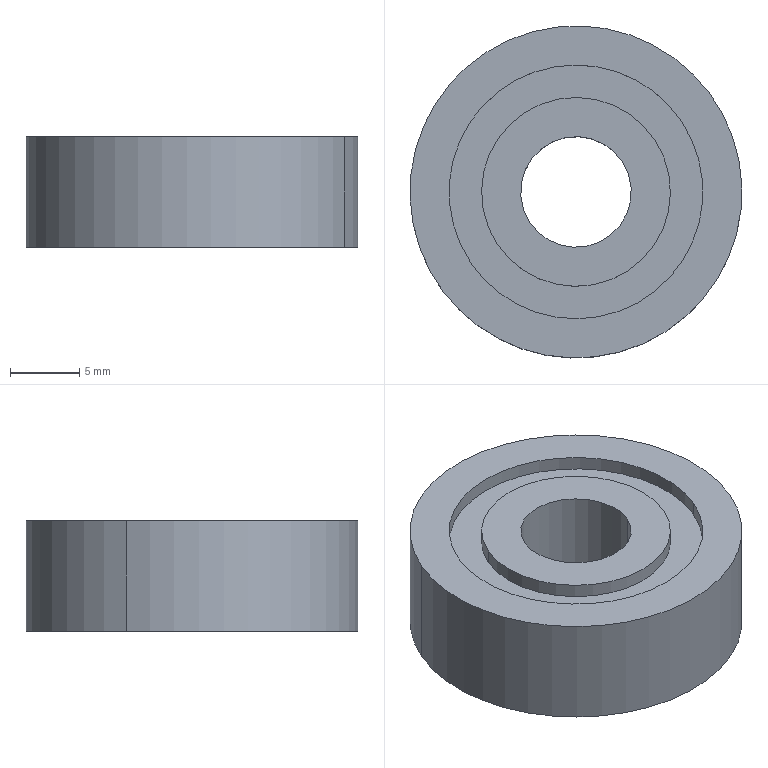Component | SolidWorks | PulleyAssembly-1_Bearing-1 | 1 solid | 18 faces | box 24 x 24 x 8 mm | volume 2981 mm3 | cylinder 12 | plane 6 | commonest cylinder face diameters 13.655 x4 18.345 x4 24 x2 8 x2
build123d program:
from build123d import *


with BuildPart() as part:
    # Sketch1 → Revolve1 (revolve)
    with BuildSketch(Plane(origin=(0, 0, 0), x_dir=(1, 0, 0), z_dir=(0, 1, 0)), mode=Mode.PRIVATE) as revolve1_sk:
        Polygon((4, 4), (6.827, 4), (6.827, 3), (9.173, 3), (9.173, 4), (12, 4), (12, -4), (9.173, -4), (9.173, -3), (6.827, -3), (6.827, -4), (4, -4), align=None)
    revolve(revolve1_sk.sketch.rotate(Axis((0, 0, -4.4), (0, 0, 1)), 180), axis=Axis((0, 0, -4.4), (0, 0, 1)))


solid = part.part

# Placed as in the assembly
solid = solid.moved(Location((-354.55, -345.434, 489.481), (0, 0, 0)))
STEP:
#1=COLOUR_RGB('',0.7922,0.8196,0.9333);
#2=FILL_AREA_STYLE_COLOUR('',#1);
#3=FILL_AREA_STYLE('',(#2));
#4=SURFACE_STYLE_FILL_AREA(#3);
#5=SURFACE_SIDE_STYLE('',(#4));
#6=SURFACE_STYLE_USAGE(.BOTH.,#5);
#7=PRESENTATION_STYLE_ASSIGNMENT((#6));
#8=CARTESIAN_POINT('',(-14.206,-13.493,19.113));
#9=VERTEX_POINT('',#8);
#10=CARTESIAN_POINT('',(-13.712,-13.706,19.113));
#11=VERTEX_POINT('',#10);
#12=CARTESIAN_POINT('',(-13.959,-13.6,19.113));
#13=DIRECTION('',(-0.,0.,1.));
#14=DIRECTION('',(-0.9185,0.3954,0.));
#15=AXIS2_PLACEMENT_3D('',#12,#13,#14);
#16=CIRCLE('',#15,0.2688);
#17=EDGE_CURVE('',#9,#11,#16,.T.);
#18=ORIENTED_EDGE('',*,*,#17,.T.);
#19=CARTESIAN_POINT('',(-13.712,-13.706,19.153));
#20=VERTEX_POINT('',#19);
#21=CARTESIAN_POINT('',(-13.712,-13.706,19.444));
#22=DIRECTION('',(-0.,0.,1.));
#23=VECTOR('',#22,39.37);
#24=LINE('',#21,#23);
#25=EDGE_CURVE('',#11,#20,#24,.T.);
#26=ORIENTED_EDGE('',*,*,#25,.T.);
#27=CARTESIAN_POINT('',(-14.206,-13.493,19.153));
#28=VERTEX_POINT('',#27);
#29=CARTESIAN_POINT('',(-13.959,-13.6,19.153));
#30=DIRECTION('',(-0.,0.,1.));
#31=DIRECTION('',(-0.9185,0.3954,0.));
#32=AXIS2_PLACEMENT_3D('',#29,#30,#31);
#33=CIRCLE('',#32,0.2688);
#34=EDGE_CURVE('',#28,#20,#33,.T.);
#35=ORIENTED_EDGE('',*,*,#34,.F.);
#36=CARTESIAN_POINT('',(-14.206,-13.493,19.444));
#37=DIRECTION('',(-0.,0.,1.));
#38=VECTOR('',#37,39.37);
#39=LINE('',#36,#38);
#40=EDGE_CURVE('',#9,#28,#39,.T.);
#41=ORIENTED_EDGE('',*,*,#40,.F.);
#42=EDGE_LOOP('',(#18,#26,#35,#41));
#43=FACE_OUTER_BOUND('',#42,.T.);
#44=CARTESIAN_POINT('',(-13.959,-13.6,19.444));
#45=DIRECTION('',(-0.,0.,1.));
#46=DIRECTION('',(-0.9185,0.3954,0.));
#47=AXIS2_PLACEMENT_3D('',#44,#45,#46);
#48=CYLINDRICAL_SURFACE('',#47,0.2688);
#49=ADVANCED_FACE('',(#43),#48,.T.);
#50=CARTESIAN_POINT('',(-13.627,-13.743,19.113));
#51=VERTEX_POINT('',#50);
#52=CARTESIAN_POINT('',(-14.29,-13.457,19.113));
#53=VERTEX_POINT('',#52);
#54=CARTESIAN_POINT('',(-13.959,-13.6,19.113));
#55=DIRECTION('',(-0.,0.,1.));
#56=DIRECTION('',(-0.9185,0.3954,0.));
#57=AXIS2_PLACEMENT_3D('',#54,#55,#56);
#58=CIRCLE('',#57,0.3611);
#59=EDGE_CURVE('',#51,#53,#58,.T.);
#60=ORIENTED_EDGE('',*,*,#59,.F.);
#61=CARTESIAN_POINT('',(-13.627,-13.743,19.153));
#62=VERTEX_POINT('',#61);
#63=CARTESIAN_POINT('',(-13.627,-13.743,19.444));
#64=DIRECTION('',(-0.,0.,1.));
#65=VECTOR('',#64,39.37);
#66=LINE('',#63,#65);
#67=EDGE_CURVE('',#51,#62,#66,.T.);
#68=ORIENTED_EDGE('',*,*,#67,.T.);
#69=CARTESIAN_POINT('',(-14.29,-13.457,19.153));
#70=VERTEX_POINT('',#69);
#71=CARTESIAN_POINT('',(-13.959,-13.6,19.153));
#72=DIRECTION('',(-0.,0.,1.));
#73=DIRECTION('',(-0.9185,0.3954,0.));
#74=AXIS2_PLACEMENT_3D('',#71,#72,#73);
#75=CIRCLE('',#74,0.3611);
#76=EDGE_CURVE('',#62,#70,#75,.T.);
#77=ORIENTED_EDGE('',*,*,#76,.T.);
#78=CARTESIAN_POINT('',(-14.29,-13.457,19.444));
#79=DIRECTION('',(-0.,0.,1.));
#80=VECTOR('',#79,39.37);
#81=LINE('',#78,#80);
#82=EDGE_CURVE('',#53,#70,#81,.T.);
#83=ORIENTED_EDGE('',*,*,#82,.F.);
#84=EDGE_LOOP('',(#60,#68,#77,#83));
#85=FACE_OUTER_BOUND('',#84,.T.);
#86=CARTESIAN_POINT('',(-13.959,-13.6,19.444));
#87=DIRECTION('',(-0.,0.,1.));
#88=DIRECTION('',(-0.9185,0.3954,0.));
#89=AXIS2_PLACEMENT_3D('',#86,#87,#88);
#90=CYLINDRICAL_SURFACE('',#89,0.3611);
#91=ADVANCED_FACE('',(#85),#90,.F.);
#92=CARTESIAN_POINT('',(-14.393,-13.413,19.113));
#93=VERTEX_POINT('',#92);
#94=CARTESIAN_POINT('',(-13.525,-13.787,19.113));
#95=VERTEX_POINT('',#94);
#96=CARTESIAN_POINT('',(-13.959,-13.6,19.113));
#97=DIRECTION('',(-0.,0.,1.));
#98=DIRECTION('',(-0.9185,0.3954,0.));
#99=AXIS2_PLACEMENT_3D('',#96,#97,#98);
#100=CIRCLE('',#99,0.4724);
#101=EDGE_CURVE('',#93,#95,#100,.T.);
#102=ORIENTED_EDGE('',*,*,#101,.T.);
#103=CARTESIAN_POINT('',(-13.525,-13.787,19.428));
#104=VERTEX_POINT('',#103);
#105=CARTESIAN_POINT('',(-13.525,-13.787,19.444));
#106=DIRECTION('',(-0.,0.,1.));
#107=VECTOR('',#106,39.37);
#108=LINE('',#105,#107);
#109=EDGE_CURVE('',#95,#104,#108,.T.);
#110=ORIENTED_EDGE('',*,*,#109,.T.);
#111=CARTESIAN_POINT('',(-14.393,-13.413,19.428));
#112=VERTEX_POINT('',#111);
#113=CARTESIAN_POINT('',(-13.959,-13.6,19.428));
#114=DIRECTION('',(-0.,0.,1.));
#115=DIRECTION('',(-0.9185,0.3954,0.));
#116=AXIS2_PLACEMENT_3D('',#113,#114,#115);
#117=CIRCLE('',#116,0.4724);
#118=EDGE_CURVE('',#112,#104,#117,.T.);
#119=ORIENTED_EDGE('',*,*,#118,.F.);
#120=CARTESIAN_POINT('',(-14.393,-13.413,19.444));
#121=DIRECTION('',(-0.,0.,1.));
#122=VECTOR('',#121,39.37);
#123=LINE('',#120,#122);
#124=EDGE_CURVE('',#93,#112,#123,.T.);
#125=ORIENTED_EDGE('',*,*,#124,.F.);
#126=EDGE_LOOP('',(#102,#110,#119,#125));
#127=FACE_OUTER_BOUND('',#126,.T.);
#128=CARTESIAN_POINT('',(-13.959,-13.6,19.444));
#129=DIRECTION('',(-0.,0.,1.));
#130=DIRECTION('',(-0.9185,0.3954,0.));
#131=AXIS2_PLACEMENT_3D('',#128,#129,#130);
#132=CYLINDRICAL_SURFACE('',#131,0.4724);
#133=ADVANCED_FACE('',(#127),#132,.T.);
#134=CARTESIAN_POINT('',(-13.627,-13.743,19.389));
#135=VERTEX_POINT('',#134);
#136=CARTESIAN_POINT('',(-14.29,-13.457,19.389));
#137=VERTEX_POINT('',#136);
#138=CARTESIAN_POINT('',(-13.959,-13.6,19.389));
#139=DIRECTION('',(-0.,0.,1.));
#140=DIRECTION('',(-0.9185,0.3954,0.));
#141=AXIS2_PLACEMENT_3D('',#138,#139,#140);
#142=CIRCLE('',#141,0.3611);
#143=EDGE_CURVE('',#135,#137,#142,.T.);
#144=ORIENTED_EDGE('',*,*,#143,.F.);
#145=CARTESIAN_POINT('',(-13.627,-13.743,19.428));
#146=VERTEX_POINT('',#145);
#147=CARTESIAN_POINT('',(-13.627,-13.743,19.444));
#148=DIRECTION('',(-0.,0.,1.));
#149=VECTOR('',#148,39.37);
#150=LINE('',#147,#149);
#151=EDGE_CURVE('',#135,#146,#150,.T.);
#152=ORIENTED_EDGE('',*,*,#151,.T.);
#153=CARTESIAN_POINT('',(-14.29,-13.457,19.428));
#154=VERTEX_POINT('',#153);
#155=CARTESIAN_POINT('',(-13.959,-13.6,19.428));
#156=DIRECTION('',(-0.,0.,1.));
#157=DIRECTION('',(-0.9185,0.3954,0.));
#158=AXIS2_PLACEMENT_3D('',#155,#156,#157);
#159=CIRCLE('',#158,0.3611);
#160=EDGE_CURVE('',#146,#154,#159,.T.);
#161=ORIENTED_EDGE('',*,*,#160,.T.);
#162=CARTESIAN_POINT('',(-14.29,-13.457,19.444));
#163=DIRECTION('',(-0.,0.,1.));
#164=VECTOR('',#163,39.37);
#165=LINE('',#162,#164);
#166=EDGE_CURVE('',#137,#154,#165,.T.);
#167=ORIENTED_EDGE('',*,*,#166,.F.);
#168=EDGE_LOOP('',(#144,#152,#161,#167));
#169=FACE_OUTER_BOUND('',#168,.T.);
#170=CARTESIAN_POINT('',(-13.959,-13.6,19.444));
#171=DIRECTION('',(-0.,0.,1.));
#172=DIRECTION('',(-0.9185,0.3954,0.));
#173=AXIS2_PLACEMENT_3D('',#170,#171,#172);
#174=CYLINDRICAL_SURFACE('',#173,0.3611);
#175=ADVANCED_FACE('',(#169),#174,.F.);
#176=CARTESIAN_POINT('',(-14.206,-13.493,19.389));
#177=VERTEX_POINT('',#176);
#178=CARTESIAN_POINT('',(-13.712,-13.706,19.389));
#179=VERTEX_POINT('',#178);
#180=CARTESIAN_POINT('',(-13.959,-13.6,19.389));
#181=DIRECTION('',(-0.,0.,1.));
#182=DIRECTION('',(-0.9185,0.3954,0.));
#183=AXIS2_PLACEMENT_3D('',#180,#181,#182);
#184=CIRCLE('',#183,0.2688);
#185=EDGE_CURVE('',#177,#179,#184,.T.);
#186=ORIENTED_EDGE('',*,*,#185,.T.);
#187=CARTESIAN_POINT('',(-13.712,-13.706,19.428));
#188=VERTEX_POINT('',#187);
#189=CARTESIAN_POINT('',(-13.712,-13.706,19.444));
#190=DIRECTION('',(-0.,0.,1.));
#191=VECTOR('',#190,39.37);
#192=LINE('',#189,#191);
#193=EDGE_CURVE('',#179,#188,#192,.T.);
#194=ORIENTED_EDGE('',*,*,#193,.T.);
#195=CARTESIAN_POINT('',(-14.206,-13.493,19.428));
#196=VERTEX_POINT('',#195);
#197=CARTESIAN_POINT('',(-13.959,-13.6,19.428));
#198=DIRECTION('',(-0.,0.,1.));
#199=DIRECTION('',(-0.9185,0.3954,0.));
#200=AXIS2_PLACEMENT_3D('',#197,#198,#199);
#201=CIRCLE('',#200,0.2688);
#202=EDGE_CURVE('',#196,#188,#201,.T.);
#203=ORIENTED_EDGE('',*,*,#202,.F.);
#204=CARTESIAN_POINT('',(-14.206,-13.493,19.444));
#205=DIRECTION('',(-0.,0.,1.));
#206=VECTOR('',#205,39.37);
#207=LINE('',#204,#206);
#208=EDGE_CURVE('',#177,#196,#207,.T.);
#209=ORIENTED_EDGE('',*,*,#208,.F.);
#210=EDGE_LOOP('',(#186,#194,#203,#209));
#211=FACE_OUTER_BOUND('',#210,.T.);
#212=CARTESIAN_POINT('',(-13.959,-13.6,19.444));
#213=DIRECTION('',(-0.,0.,1.));
#214=DIRECTION('',(-0.9185,0.3954,0.));
#215=AXIS2_PLACEMENT_3D('',#212,#213,#214);
#216=CYLINDRICAL_SURFACE('',#215,0.2688);
#217=ADVANCED_FACE('',(#211),#216,.T.);
#218=CARTESIAN_POINT('',(-13.814,-13.662,19.113));
#219=VERTEX_POINT('',#218);
#220=CARTESIAN_POINT('',(-14.103,-13.537,19.113));
#221=VERTEX_POINT('',#220);
#222=CARTESIAN_POINT('',(-13.959,-13.6,19.113));
#223=DIRECTION('',(-0.,0.,1.));
#224=DIRECTION('',(-0.9185,0.3954,0.));
#225=AXIS2_PLACEMENT_3D('',#222,#223,#224);
#226=CIRCLE('',#225,0.1575);
#227=EDGE_CURVE('',#219,#221,#226,.T.);
#228=ORIENTED_EDGE('',*,*,#227,.F.);
#229=CARTESIAN_POINT('',(-13.814,-13.662,19.428));
#230=VERTEX_POINT('',#229);
#231=CARTESIAN_POINT('',(-13.814,-13.662,19.444));
#232=DIRECTION('',(-0.,0.,1.));
#233=VECTOR('',#232,39.37);
#234=LINE('',#231,#233);
#235=EDGE_CURVE('',#219,#230,#234,.T.);
#236=ORIENTED_EDGE('',*,*,#235,.T.);
#237=CARTESIAN_POINT('',(-14.103,-13.537,19.428));
#238=VERTEX_POINT('',#237);
#239=CARTESIAN_POINT('',(-13.959,-13.6,19.428));
#240=DIRECTION('',(-0.,0.,1.));
#241=DIRECTION('',(-0.9185,0.3954,0.));
#242=AXIS2_PLACEMENT_3D('',#239,#240,#241);
#243=CIRCLE('',#242,0.1575);
#244=EDGE_CURVE('',#230,#238,#243,.T.);
#245=ORIENTED_EDGE('',*,*,#244,.T.);
#246=CARTESIAN_POINT('',(-14.103,-13.537,19.444));
#247=DIRECTION('',(-0.,0.,1.));
#248=VECTOR('',#247,39.37);
#249=LINE('',#246,#248);
#250=EDGE_CURVE('',#221,#238,#249,.T.);
#251=ORIENTED_EDGE('',*,*,#250,.F.);
#252=EDGE_LOOP('',(#228,#236,#245,#251));
#253=FACE_OUTER_BOUND('',#252,.T.);
#254=CARTESIAN_POINT('',(-13.959,-13.6,19.444));
#255=DIRECTION('',(-0.,0.,1.));
#256=DIRECTION('',(-0.9185,0.3954,0.));
#257=AXIS2_PLACEMENT_3D('',#254,#255,#256);
#258=CYLINDRICAL_SURFACE('',#257,0.1575);
#259=ADVANCED_FACE('',(#253),#258,.F.);
#260=ORIENTED_EDGE('',*,*,#235,.F.);
#261=CARTESIAN_POINT('',(-13.959,-13.6,19.113));
#262=DIRECTION('',(-0.,0.,1.));
#263=DIRECTION('',(-0.9185,0.3954,0.));
#264=AXIS2_PLACEMENT_3D('',#261,#262,#263);
#265=CIRCLE('',#264,0.1575);
#266=EDGE_CURVE('',#221,#219,#265,.T.);
#267=ORIENTED_EDGE('',*,*,#266,.F.);
#268=ORIENTED_EDGE('',*,*,#250,.T.);
#269=CARTESIAN_POINT('',(-13.959,-13.6,19.428));
#270=DIRECTION('',(-0.,0.,1.));
#271=DIRECTION('',(-0.9185,0.3954,0.));
#272=AXIS2_PLACEMENT_3D('',#269,#270,#271);
#273=CIRCLE('',#272,0.1575);
#274=EDGE_CURVE('',#238,#230,#273,.T.);
#275=ORIENTED_EDGE('',*,*,#274,.T.);
#276=EDGE_LOOP('',(#260,#267,#268,#275));
#277=FACE_OUTER_BOUND('',#276,.T.);
#278=CARTESIAN_POINT('',(-13.959,-13.6,19.444));
#279=DIRECTION('',(-0.,0.,1.));
#280=DIRECTION('',(-0.9185,0.3954,0.));
#281=AXIS2_PLACEMENT_3D('',#278,#279,#280);
#282=CYLINDRICAL_SURFACE('',#281,0.1575);
#283=ADVANCED_FACE('',(#277),#282,.F.);
#284=ORIENTED_EDGE('',*,*,#274,.F.);
#285=ORIENTED_EDGE('',*,*,#244,.F.);
#286=EDGE_LOOP('',(#284,#285));
#287=FACE_BOUND('',#286,.T.);
#288=ORIENTED_EDGE('',*,*,#202,.T.);
#289=CARTESIAN_POINT('',(-13.959,-13.6,19.428));
#290=DIRECTION('',(-0.,0.,1.));
#291=DIRECTION('',(-0.9185,0.3954,0.));
#292=AXIS2_PLACEMENT_3D('',#289,#290,#291);
#293=CIRCLE('',#292,0.2688);
#294=EDGE_CURVE('',#188,#196,#293,.T.);
#295=ORIENTED_EDGE('',*,*,#294,.T.);
#296=EDGE_LOOP('',(#288,#295));
#297=FACE_OUTER_BOUND('',#296,.T.);
#298=CARTESIAN_POINT('',(-13.814,-13.662,19.428));
#299=DIRECTION('',(0.,-0.,-1.));
#300=DIRECTION('',(0.9185,-0.3954,0.));
#301=AXIS2_PLACEMENT_3D('',#298,#299,#300);
#302=PLANE('',#301);
#303=ADVANCED_FACE('',(#287,#297),#302,.F.);
#304=ORIENTED_EDGE('',*,*,#193,.F.);
#305=CARTESIAN_POINT('',(-13.959,-13.6,19.389));
#306=DIRECTION('',(-0.,0.,1.));
#307=DIRECTION('',(-0.9185,0.3954,0.));
#308=AXIS2_PLACEMENT_3D('',#305,#306,#307);
#309=CIRCLE('',#308,0.2688);
#310=EDGE_CURVE('',#179,#177,#309,.T.);
#311=ORIENTED_EDGE('',*,*,#310,.T.);
#312=ORIENTED_EDGE('',*,*,#208,.T.);
#313=ORIENTED_EDGE('',*,*,#294,.F.);
#314=EDGE_LOOP('',(#304,#311,#312,#313));
#315=FACE_OUTER_BOUND('',#314,.T.);
#316=CARTESIAN_POINT('',(-13.959,-13.6,19.444));
#317=DIRECTION('',(-0.,0.,1.));
#318=DIRECTION('',(-0.9185,0.3954,0.));
#319=AXIS2_PLACEMENT_3D('',#316,#317,#318);
#320=CYLINDRICAL_SURFACE('',#319,0.2688);
#321=ADVANCED_FACE('',(#315),#320,.T.);
#322=ORIENTED_EDGE('',*,*,#185,.F.);
#323=ORIENTED_EDGE('',*,*,#310,.F.);
#324=EDGE_LOOP('',(#322,#323));
#325=FACE_BOUND('',#324,.T.);
#326=CARTESIAN_POINT('',(-13.959,-13.6,19.389));
#327=DIRECTION('',(-0.,0.,1.));
#328=DIRECTION('',(-0.9185,0.3954,0.));
#329=AXIS2_PLACEMENT_3D('',#326,#327,#328);
#330=CIRCLE('',#329,0.3611);
#331=EDGE_CURVE('',#137,#135,#330,.T.);
#332=ORIENTED_EDGE('',*,*,#331,.T.);
#333=ORIENTED_EDGE('',*,*,#143,.T.);
#334=EDGE_LOOP('',(#332,#333));
#335=FACE_OUTER_BOUND('',#334,.T.);
#336=CARTESIAN_POINT('',(-13.627,-13.743,19.389));
#337=DIRECTION('',(0.,-0.,-1.));
#338=DIRECTION('',(0.9185,-0.3954,0.));
#339=AXIS2_PLACEMENT_3D('',#336,#337,#338);
#340=PLANE('',#339);
#341=ADVANCED_FACE('',(#325,#335),#340,.F.);
#342=ORIENTED_EDGE('',*,*,#151,.F.);
#343=ORIENTED_EDGE('',*,*,#331,.F.);
#344=ORIENTED_EDGE('',*,*,#166,.T.);
#345=CARTESIAN_POINT('',(-13.959,-13.6,19.428));
#346=DIRECTION('',(-0.,0.,1.));
#347=DIRECTION('',(-0.9185,0.3954,0.));
#348=AXIS2_PLACEMENT_3D('',#345,#346,#347);
#349=CIRCLE('',#348,0.3611);
#350=EDGE_CURVE('',#154,#146,#349,.T.);
#351=ORIENTED_EDGE('',*,*,#350,.T.);
#352=EDGE_LOOP('',(#342,#343,#344,#351));
#353=FACE_OUTER_BOUND('',#352,.T.);
#354=CARTESIAN_POINT('',(-13.959,-13.6,19.444));
#355=DIRECTION('',(-0.,0.,1.));
#356=DIRECTION('',(-0.9185,0.3954,0.));
#357=AXIS2_PLACEMENT_3D('',#354,#355,#356);
#358=CYLINDRICAL_SURFACE('',#357,0.3611);
#359=ADVANCED_FACE('',(#353),#358,.F.);
#360=ORIENTED_EDGE('',*,*,#350,.F.);
#361=ORIENTED_EDGE('',*,*,#160,.F.);
#362=EDGE_LOOP('',(#360,#361));
#363=FACE_BOUND('',#362,.T.);
#364=ORIENTED_EDGE('',*,*,#118,.T.);
#365=CARTESIAN_POINT('',(-13.959,-13.6,19.428));
#366=DIRECTION('',(-0.,0.,1.));
#367=DIRECTION('',(-0.9185,0.3954,0.));
#368=AXIS2_PLACEMENT_3D('',#365,#366,#367);
#369=CIRCLE('',#368,0.4724);
#370=EDGE_CURVE('',#104,#112,#369,.T.);
#371=ORIENTED_EDGE('',*,*,#370,.T.);
#372=EDGE_LOOP('',(#364,#371));
#373=FACE_OUTER_BOUND('',#372,.T.);
#374=CARTESIAN_POINT('',(-13.627,-13.743,19.428));
#375=DIRECTION('',(0.,-0.,-1.));
#376=DIRECTION('',(0.9185,-0.3954,0.));
#377=AXIS2_PLACEMENT_3D('',#374,#375,#376);
#378=PLANE('',#377);
#379=ADVANCED_FACE('',(#363,#373),#378,.F.);
#380=ORIENTED_EDGE('',*,*,#109,.F.);
#381=CARTESIAN_POINT('',(-13.959,-13.6,19.113));
#382=DIRECTION('',(-0.,0.,1.));
#383=DIRECTION('',(-0.9185,0.3954,0.));
#384=AXIS2_PLACEMENT_3D('',#381,#382,#383);
#385=CIRCLE('',#384,0.4724);
#386=EDGE_CURVE('',#95,#93,#385,.T.);
#387=ORIENTED_EDGE('',*,*,#386,.T.);
#388=ORIENTED_EDGE('',*,*,#124,.T.);
#389=ORIENTED_EDGE('',*,*,#370,.F.);
#390=EDGE_LOOP('',(#380,#387,#388,#389));
#391=FACE_OUTER_BOUND('',#390,.T.);
#392=CARTESIAN_POINT('',(-13.959,-13.6,19.444));
#393=DIRECTION('',(-0.,0.,1.));
#394=DIRECTION('',(-0.9185,0.3954,0.));
#395=AXIS2_PLACEMENT_3D('',#392,#393,#394);
#396=CYLINDRICAL_SURFACE('',#395,0.4724);
#397=ADVANCED_FACE('',(#391),#396,.T.);
#398=ORIENTED_EDGE('',*,*,#101,.F.);
#399=ORIENTED_EDGE('',*,*,#386,.F.);
#400=EDGE_LOOP('',(#398,#399));
#401=FACE_OUTER_BOUND('',#400,.T.);
#402=CARTESIAN_POINT('',(-13.959,-13.6,19.113));
#403=DIRECTION('',(-0.,0.,1.));
#404=DIRECTION('',(-0.9185,0.3954,0.));
#405=AXIS2_PLACEMENT_3D('',#402,#403,#404);
#406=CIRCLE('',#405,0.3611);
#407=EDGE_CURVE('',#53,#51,#406,.T.);
#408=ORIENTED_EDGE('',*,*,#407,.T.);
#409=ORIENTED_EDGE('',*,*,#59,.T.);
#410=EDGE_LOOP('',(#408,#409));
#411=FACE_BOUND('',#410,.T.);
#412=CARTESIAN_POINT('',(-13.525,-13.787,19.113));
#413=DIRECTION('',(-0.,0.,1.));
#414=DIRECTION('',(-0.9185,0.3954,-0.));
#415=AXIS2_PLACEMENT_3D('',#412,#413,#414);
#416=PLANE('',#415);
#417=ADVANCED_FACE('',(#401,#411),#416,.F.);
#418=ORIENTED_EDGE('',*,*,#67,.F.);
#419=ORIENTED_EDGE('',*,*,#407,.F.);
#420=ORIENTED_EDGE('',*,*,#82,.T.);
#421=CARTESIAN_POINT('',(-13.959,-13.6,19.153));
#422=DIRECTION('',(-0.,0.,1.));
#423=DIRECTION('',(-0.9185,0.3954,0.));
#424=AXIS2_PLACEMENT_3D('',#421,#422,#423);
#425=CIRCLE('',#424,0.3611);
#426=EDGE_CURVE('',#70,#62,#425,.T.);
#427=ORIENTED_EDGE('',*,*,#426,.T.);
#428=EDGE_LOOP('',(#418,#419,#420,#427));
#429=FACE_OUTER_BOUND('',#428,.T.);
#430=CARTESIAN_POINT('',(-13.959,-13.6,19.444));
#431=DIRECTION('',(-0.,0.,1.));
#432=DIRECTION('',(-0.9185,0.3954,0.));
#433=AXIS2_PLACEMENT_3D('',#430,#431,#432);
#434=CYLINDRICAL_SURFACE('',#433,0.3611);
#435=ADVANCED_FACE('',(#429),#434,.F.);
#436=ORIENTED_EDGE('',*,*,#426,.F.);
#437=ORIENTED_EDGE('',*,*,#76,.F.);
#438=EDGE_LOOP('',(#436,#437));
#439=FACE_OUTER_BOUND('',#438,.T.);
#440=ORIENTED_EDGE('',*,*,#34,.T.);
#441=CARTESIAN_POINT('',(-13.959,-13.6,19.153));
#442=DIRECTION('',(-0.,0.,1.));
#443=DIRECTION('',(-0.9185,0.3954,0.));
#444=AXIS2_PLACEMENT_3D('',#441,#442,#443);
#445=CIRCLE('',#444,0.2688);
#446=EDGE_CURVE('',#20,#28,#445,.T.);
#447=ORIENTED_EDGE('',*,*,#446,.T.);
#448=EDGE_LOOP('',(#440,#447));
#449=FACE_BOUND('',#448,.T.);
#450=CARTESIAN_POINT('',(-13.627,-13.743,19.153));
#451=DIRECTION('',(-0.,0.,1.));
#452=DIRECTION('',(-0.9185,0.3954,-0.));
#453=AXIS2_PLACEMENT_3D('',#450,#451,#452);
#454=PLANE('',#453);
#455=ADVANCED_FACE('',(#439,#449),#454,.F.);
#456=ORIENTED_EDGE('',*,*,#25,.F.);
#457=CARTESIAN_POINT('',(-13.959,-13.6,19.113));
#458=DIRECTION('',(-0.,0.,1.));
#459=DIRECTION('',(-0.9185,0.3954,0.));
#460=AXIS2_PLACEMENT_3D('',#457,#458,#459);
#461=CIRCLE('',#460,0.2688);
#462=EDGE_CURVE('',#11,#9,#461,.T.);
#463=ORIENTED_EDGE('',*,*,#462,.T.);
#464=ORIENTED_EDGE('',*,*,#40,.T.);
#465=ORIENTED_EDGE('',*,*,#446,.F.);
#466=EDGE_LOOP('',(#456,#463,#464,#465));
#467=FACE_OUTER_BOUND('',#466,.T.);
#468=CARTESIAN_POINT('',(-13.959,-13.6,19.444));
#469=DIRECTION('',(-0.,0.,1.));
#470=DIRECTION('',(-0.9185,0.3954,0.));
#471=AXIS2_PLACEMENT_3D('',#468,#469,#470);
#472=CYLINDRICAL_SURFACE('',#471,0.2688);
#473=ADVANCED_FACE('',(#467),#472,.T.);
#474=ORIENTED_EDGE('',*,*,#17,.F.);
#475=ORIENTED_EDGE('',*,*,#462,.F.);
#476=EDGE_LOOP('',(#474,#475));
#477=FACE_OUTER_BOUND('',#476,.T.);
#478=ORIENTED_EDGE('',*,*,#266,.T.);
#479=ORIENTED_EDGE('',*,*,#227,.T.);
#480=EDGE_LOOP('',(#478,#479));
#481=FACE_BOUND('',#480,.T.);
#482=CARTESIAN_POINT('',(-13.712,-13.706,19.113));
#483=DIRECTION('',(-0.,0.,1.));
#484=DIRECTION('',(-0.9185,0.3954,-0.));
#485=AXIS2_PLACEMENT_3D('',#482,#483,#484);
#486=PLANE('',#485);
#487=ADVANCED_FACE('',(#477,#481),#486,.F.);
#488=CLOSED_SHELL('',(#49,#91,#133,#175,#217,#259,#283,#303,#321,#341,#359,#379,#397,#417,#435,#455,#473,#487));
#489=MANIFOLD_SOLID_BREP('',#488);
#490=STYLED_ITEM('',(#7),#489);
#491=(LENGTH_UNIT()NAMED_UNIT(*)SI_UNIT($,.METRE.));
#492=LENGTH_MEASURE_WITH_UNIT(LENGTH_MEASURE(0.0254),#491);
#493=DIMENSIONAL_EXPONENTS(1.,0.,0.,0.,0.,0.,0.);
#494=(CONVERSION_BASED_UNIT('',#492)LENGTH_UNIT()NAMED_UNIT(#493));
#495=UNCERTAINTY_MEASURE_WITH_UNIT(LENGTH_MEASURE(0.00001),#494,'','');
#496=(NAMED_UNIT(*)PLANE_ANGLE_UNIT()SI_UNIT($,.RADIAN.));
#497=(NAMED_UNIT(*)SI_UNIT($,.STERADIAN.)SOLID_ANGLE_UNIT());
#498=(GEOMETRIC_REPRESENTATION_CONTEXT(3)GLOBAL_UNCERTAINTY_ASSIGNED_CONTEXT((#495))GLOBAL_UNIT_ASSIGNED_CONTEXT((#494,#496,#497))REPRESENTATION_CONTEXT('',''));
#499=MECHANICAL_DESIGN_GEOMETRIC_PRESENTATION_REPRESENTATION('',(#490),#498);
#500=PRESENTATION_LAYER_ASSIGNMENT('','',(#490));
#501=CARTESIAN_POINT('',(0.,0.,0.));
#502=DIRECTION('',(0.,0.,1.));
#503=DIRECTION('',(1.,0.,0.));
#504=AXIS2_PLACEMENT_3D('',#501,#502,#503);
#505=(LENGTH_UNIT()NAMED_UNIT(*)SI_UNIT($,.METRE.));
#506=LENGTH_MEASURE_WITH_UNIT(LENGTH_MEASURE(0.0254),#505);
#507=DIMENSIONAL_EXPONENTS(1.,0.,0.,0.,0.,0.,0.);
#508=(CONVERSION_BASED_UNIT('',#506)LENGTH_UNIT()NAMED_UNIT(#507));
#509=UNCERTAINTY_MEASURE_WITH_UNIT(LENGTH_MEASURE(0.00001),#508,'','');
#510=(NAMED_UNIT(*)PLANE_ANGLE_UNIT()SI_UNIT($,.RADIAN.));
#511=(NAMED_UNIT(*)SI_UNIT($,.STERADIAN.)SOLID_ANGLE_UNIT());
#512=(GEOMETRIC_REPRESENTATION_CONTEXT(3)GLOBAL_UNCERTAINTY_ASSIGNED_CONTEXT((#509))GLOBAL_UNIT_ASSIGNED_CONTEXT((#508,#510,#511))REPRESENTATION_CONTEXT('',''));
#513=ADVANCED_BREP_SHAPE_REPRESENTATION('',(#489,#504),#512);